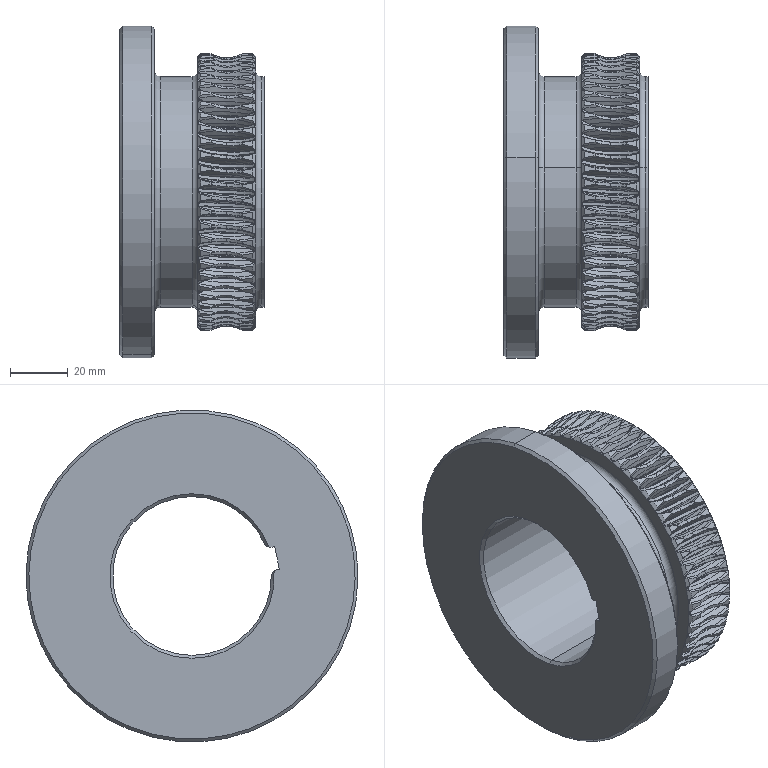Component | SolidWorks | 1Turbine-1 | 1 solid | 1545 faces | volume 211160 mm3 | spline 1260 | cylinder 133 | torus 126 | cone 14 | plane 12 | commonest cylinder face diameters 96 x120 80 x4 55 x3 86 x2 105 x2 115 x2